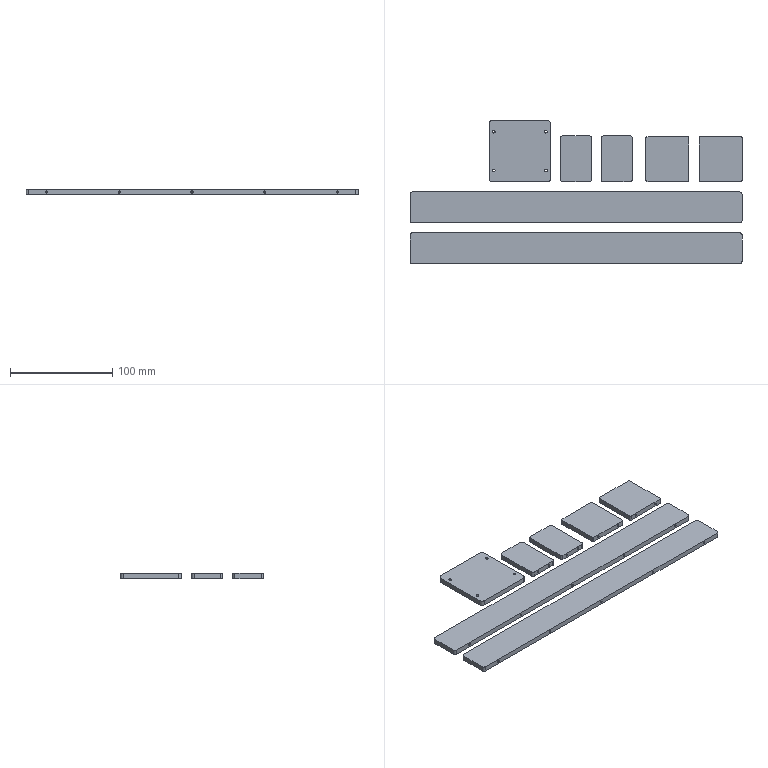CAM job | Mastercam | mm | 9 operations | part box 325 x 140 x 5
1. Contour (Ramp) | 4 - 4 平铣刀
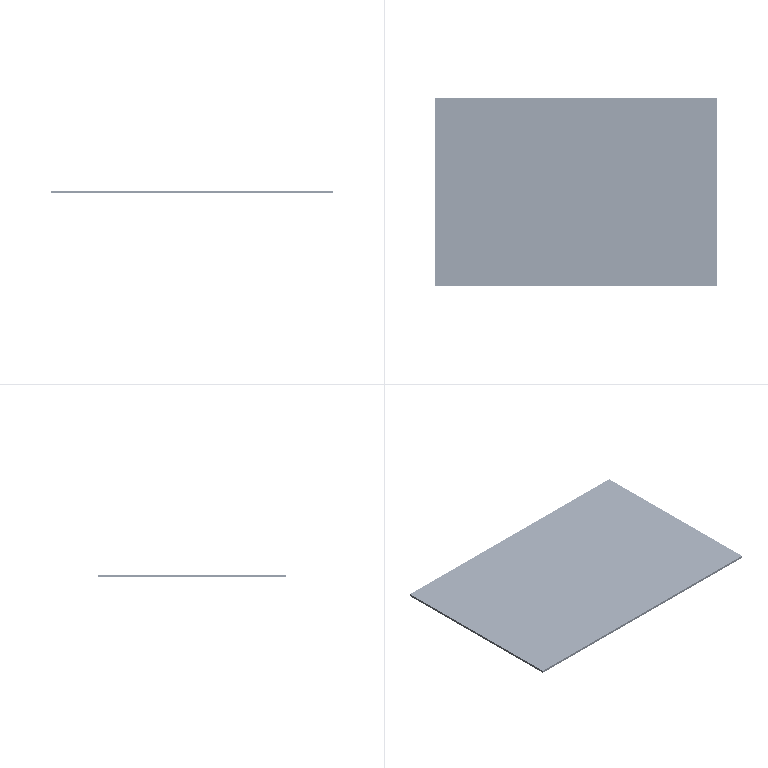2. Contour (2D chamfer) | 5 - 4 倒角刀
3. Drill/Counterbore | 5 - 4 倒角刀
4. Contour (Ramp) | 3 - 3 平铣刀
5. Drill/Counterbore | 5 - 4 倒角刀
6. Drill/Counterbore | 5 - 4 倒角刀
7. Drill/Counterbore | 5 - 4 倒角刀
8. Drill/Counterbore | 5 - 4 倒角刀
9. Drill/Counterbore | 5 - 4 倒角刀